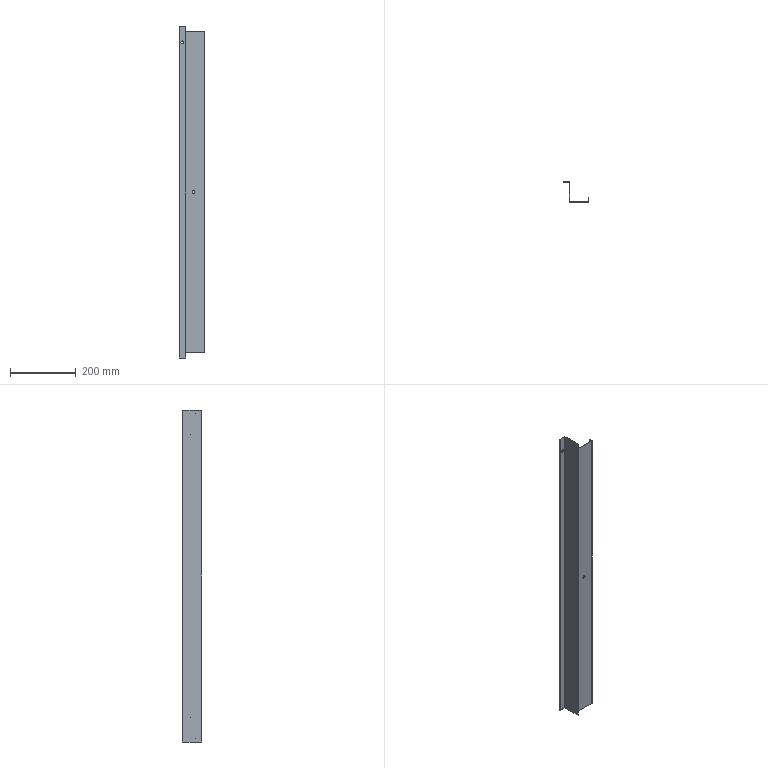Component | SolidWorks | CabinetWelding-1_FrontLowerBeam-1 | 1 solid | 48 faces | volume 176255 mm3 | plane 24 | cylinder 22 | spline 2 | commonest cylinder face diameters 0.5 x8 3 x4 9 x2 8.5 x2 0.2 x2 2.6 x2 0.4 x1 2.8 x1